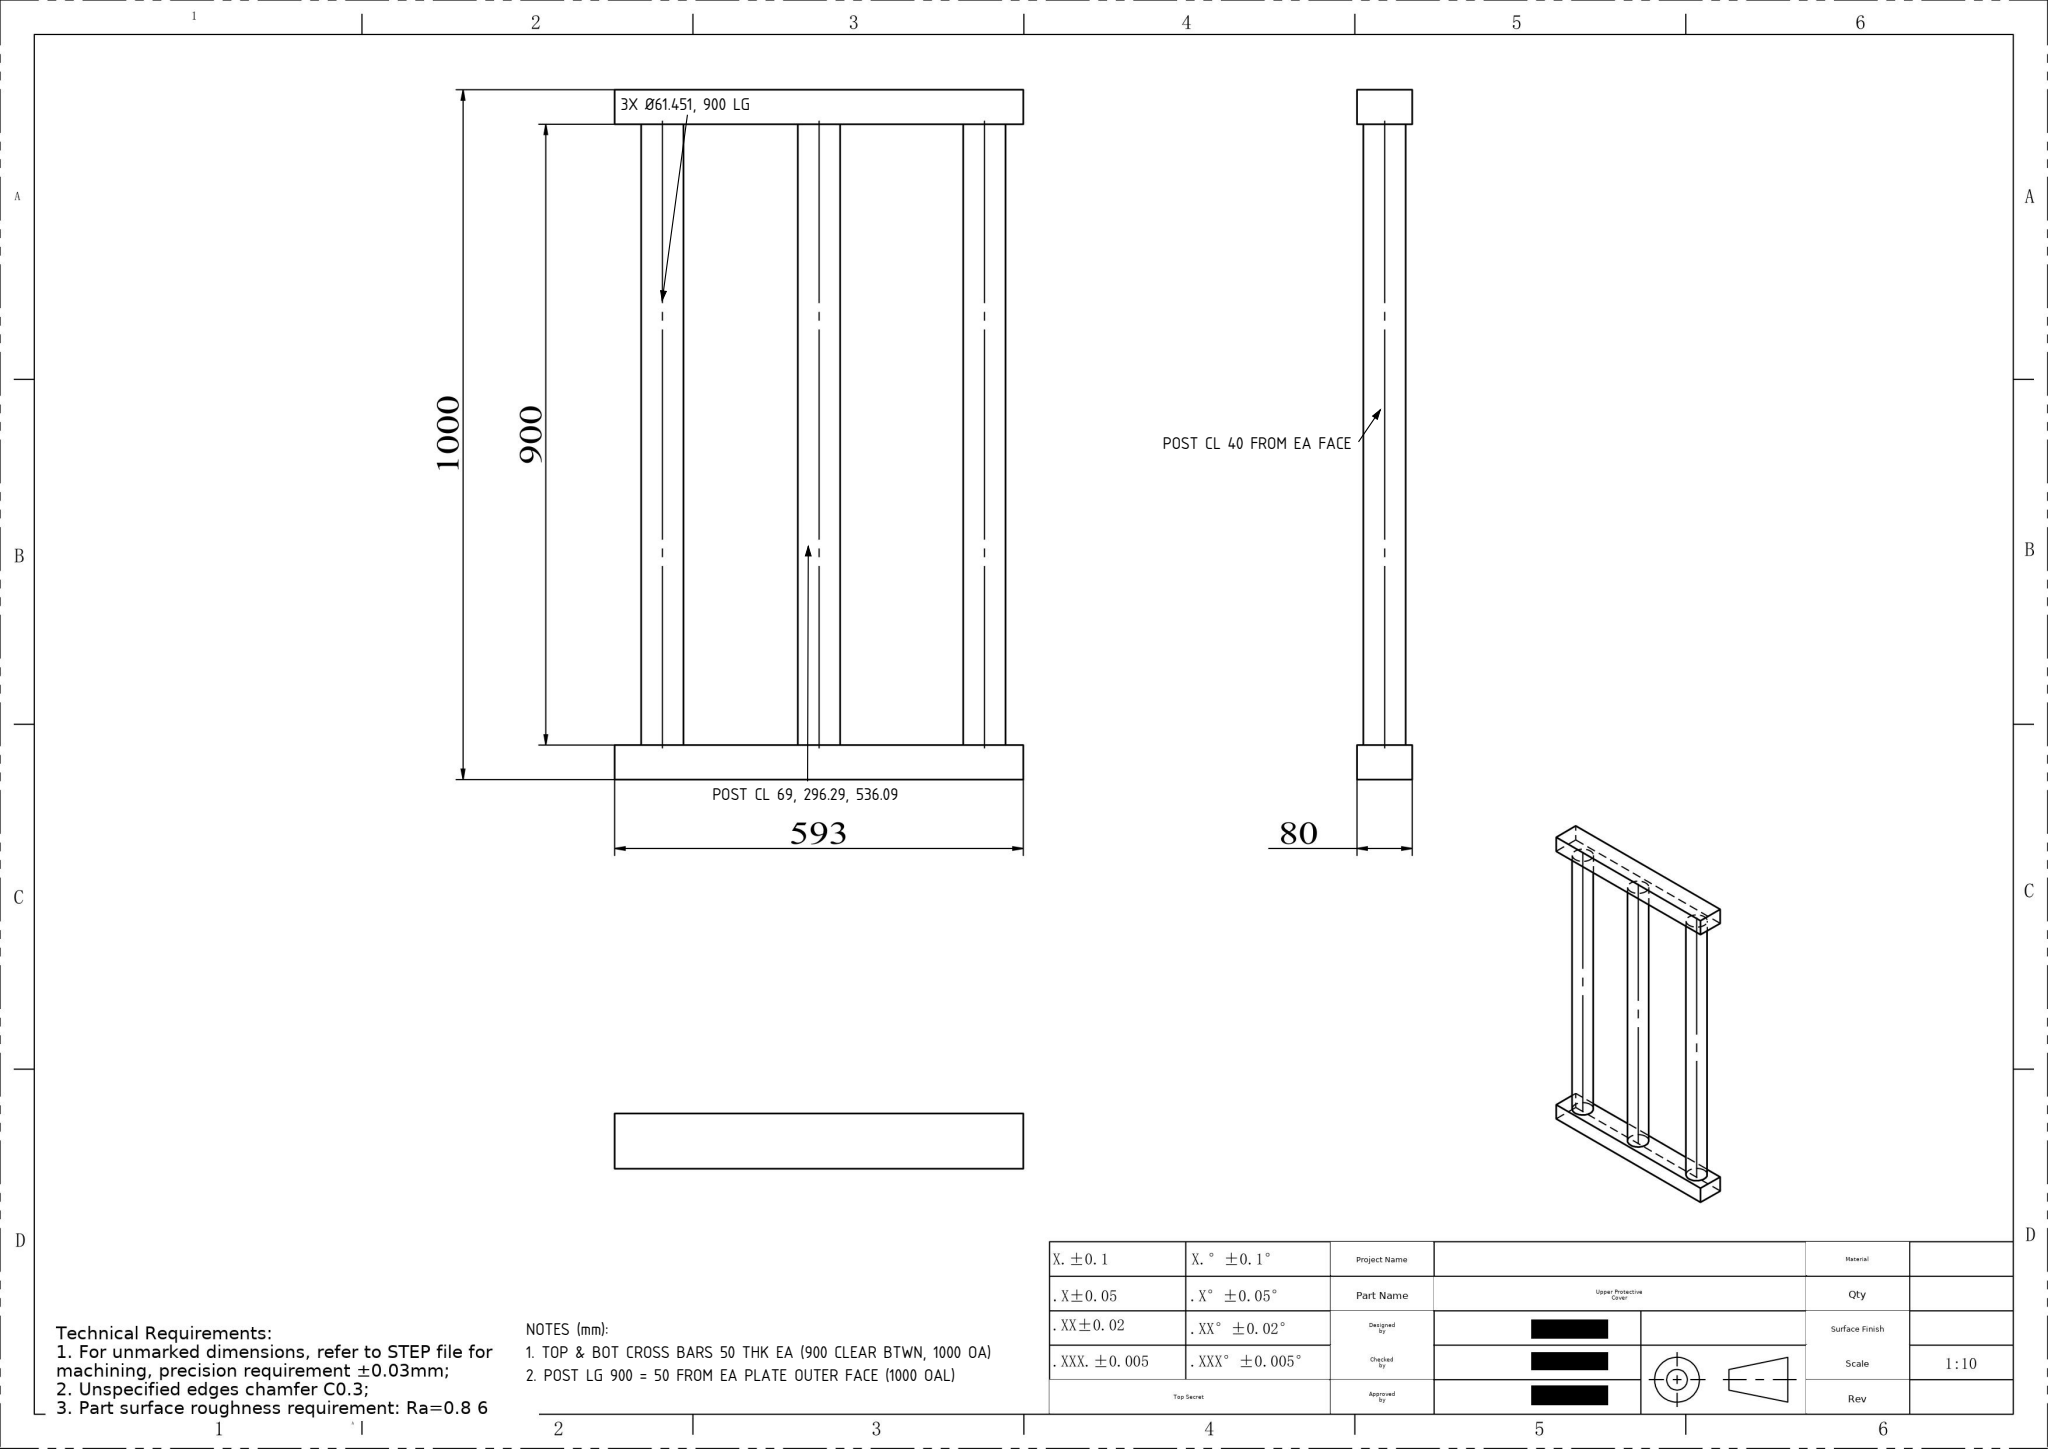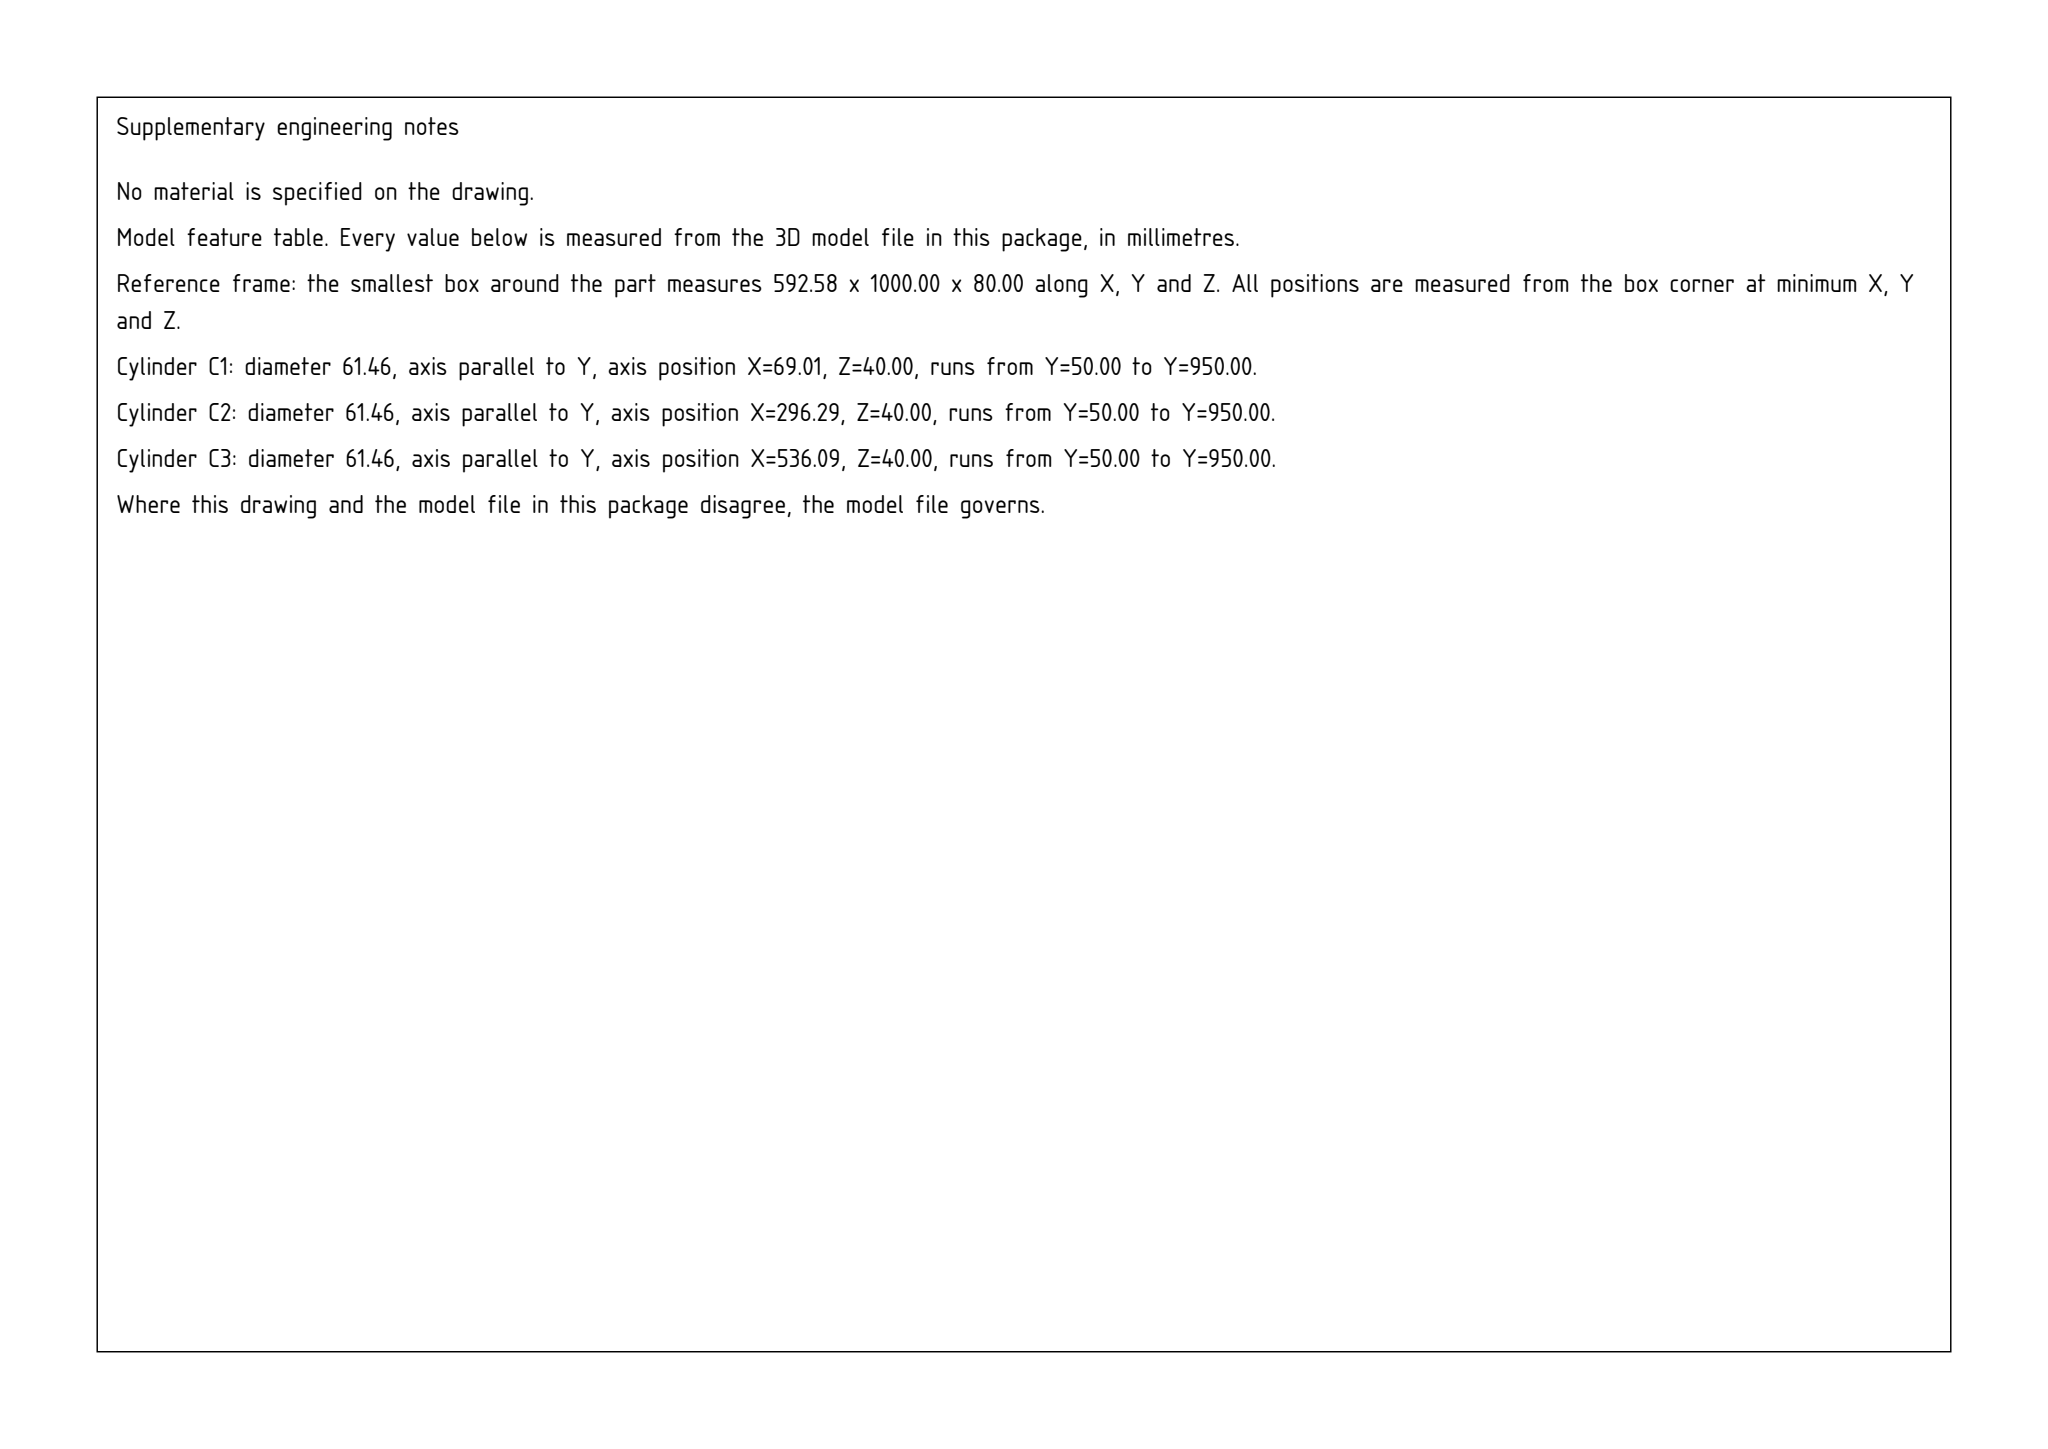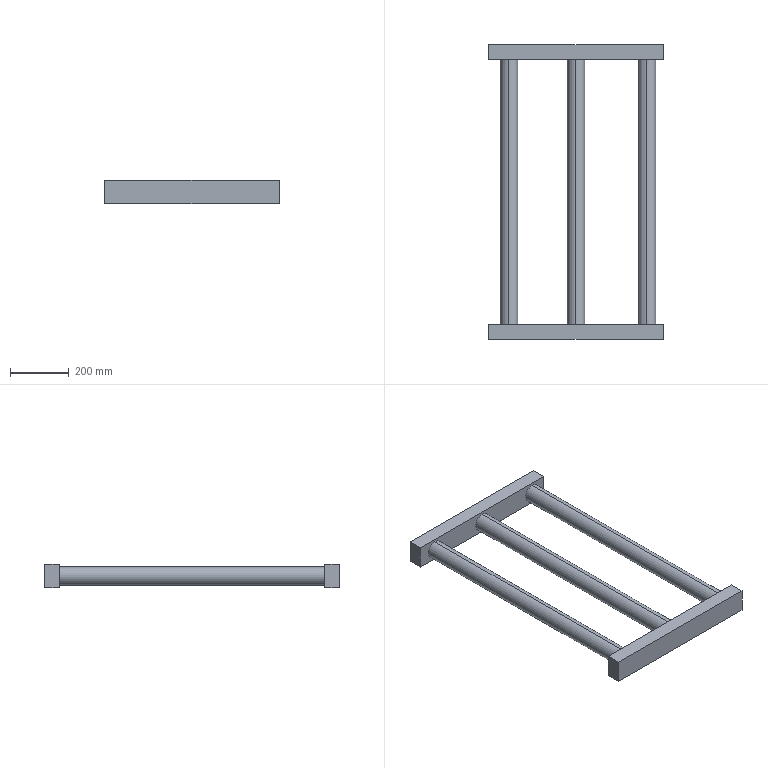Part | SolidWorks | mm | 1 solid | 18 faces | box 592.58 x 1000 x 80 mm | volume 12748485 mm3 | plane 12 | cylinder 6 | commonest cylinder face diameters 61.451 x6
Drawing notes:
TOP & BOT CROSS BARS 50 THK EA (900 CLEAR BTWN, 1000 OA) | from the solid: y-planes at 0/50 and 950/1000; rod length 900, bbox Y=1000
3X Ø61.451 VERT POSTS, 900 LG, FULL DEPTH BTWN END PLATES | from the solid: cylinders dia 61.451, axis y, length 900; plates y0-50 & y950-1000
POST CL FROM LH EDGE OF 593: 69, 296.29, 536.09 | from the solid: cylinder x positions 69.0, 296.29, 536.09 within bbox x=592.583
POST CL CENTERED IN 80 THK: 40 FROM EACH FACE | from the solid: cylinder z position 40.0; z planes at 0 and 80
POST LG 900 = 50 FROM EA PLATE OUTER FACE (1000 OAL) | from the solid: y planes 0, 50, 950, 1000; cylinder length 900
build123d program:
from build123d import *

# Parameters (mm, degrees)
SKETCH1_W             = 592.583
SKETCH1_H             = 50
BOSS_EXTRUDE1_DEPTH   = 80
BOSS_EXTRUDE1_2_DEPTH = 80
SKETCH2_R             = 30.726
BOSS_EXTRUDE2_DEPTH   = 950


with BuildPart() as part:
    # Sketch1 → Boss-Extrude1 (new body)
    with BuildSketch(Plane.XY):
        with Locations((-1944.166, 3836.21)):
            Rectangle(SKETCH1_W, SKETCH1_H)
    extrude(amount=BOSS_EXTRUDE1_DEPTH)



with BuildPart() as body_2:
    # Sketch1 → Boss-Extrude1 2 (new body)
    with BuildSketch(Plane.XY):
        with Locations((-1944.166, 2886.21)):
            Rectangle(SKETCH1_W, SKETCH1_H)
    extrude(amount=BOSS_EXTRUDE1_2_DEPTH)


with BuildPart() as part_1:
    add(part.part)

    add(body_2.part)  # Boss-Extrude2 merges body 2
    # Sketch2 → Boss-Extrude2 (add)
    with BuildSketch(Plane.XZ.offset(-3811.21)):
        with Locations(Location((-2171.453, 40, 0), (0, 0, 90))):
            Circle(SKETCH2_R)
        with Locations(Location((-1944.166, 40, 0), (0, 0, 90))):
            Circle(SKETCH2_R)
        with Locations(Location((-1704.372, 40, 0), (0, 0, 90))):
            Circle(SKETCH2_R)
    extrude(amount=BOSS_EXTRUDE2_DEPTH)


solid = part_1.part
STEP:
#1=CARTESIAN_POINT('',(-1704.372,2911.21,70.726));
#2=VERTEX_POINT('',#1);
#3=CARTESIAN_POINT('',(-1704.372,2911.21,9.274));
#4=VERTEX_POINT('',#3);
#5=CARTESIAN_POINT('',(-1704.372,2911.21,40.));
#6=DIRECTION('',(0.,1.,0.));
#7=DIRECTION('',(0.,0.,-1.));
#8=AXIS2_PLACEMENT_3D('',#5,#6,#7);
#9=CIRCLE('',#8,30.726);
#10=EDGE_CURVE('',#2,#4,#9,.T.);
#11=ORIENTED_EDGE('',*,*,#10,.T.);
#12=CARTESIAN_POINT('',(-1704.372,3811.21,9.274));
#13=VERTEX_POINT('',#12);
#14=CARTESIAN_POINT('',(-1704.372,2911.21,9.274));
#15=DIRECTION('',(0.,1.,0.));
#16=VECTOR('',#15,1000.);
#17=LINE('',#14,#16);
#18=EDGE_CURVE('',#4,#13,#17,.T.);
#19=ORIENTED_EDGE('',*,*,#18,.T.);
#20=CARTESIAN_POINT('',(-1704.372,3811.21,70.726));
#21=VERTEX_POINT('',#20);
#22=CARTESIAN_POINT('',(-1704.372,3811.21,40.));
#23=DIRECTION('',(0.,-1.,0.));
#24=DIRECTION('',(0.,0.,1.));
#25=AXIS2_PLACEMENT_3D('',#22,#23,#24);
#26=CIRCLE('',#25,30.726);
#27=EDGE_CURVE('',#13,#21,#26,.T.);
#28=ORIENTED_EDGE('',*,*,#27,.T.);
#29=CARTESIAN_POINT('',(-1704.372,2911.21,70.726));
#30=DIRECTION('',(0.,1.,0.));
#31=VECTOR('',#30,1000.);
#32=LINE('',#29,#31);
#33=EDGE_CURVE('',#2,#21,#32,.T.);
#34=ORIENTED_EDGE('',*,*,#33,.F.);
#35=EDGE_LOOP('',(#11,#19,#28,#34));
#36=FACE_OUTER_BOUND('',#35,.T.);
#37=CARTESIAN_POINT('',(-1704.372,2911.21,40.));
#38=DIRECTION('',(0.,1.,0.));
#39=DIRECTION('',(0.,0.,1.));
#40=AXIS2_PLACEMENT_3D('',#37,#38,#39);
#41=CYLINDRICAL_SURFACE('',#40,30.726);
#42=ADVANCED_FACE('',(#36),#41,.T.);
#43=CARTESIAN_POINT('',(-1944.166,2911.21,70.726));
#44=VERTEX_POINT('',#43);
#45=CARTESIAN_POINT('',(-1944.166,2911.21,9.274));
#46=VERTEX_POINT('',#45);
#47=CARTESIAN_POINT('',(-1944.166,2911.21,40.));
#48=DIRECTION('',(0.,1.,0.));
#49=DIRECTION('',(0.,0.,-1.));
#50=AXIS2_PLACEMENT_3D('',#47,#48,#49);
#51=CIRCLE('',#50,30.726);
#52=EDGE_CURVE('',#44,#46,#51,.T.);
#53=ORIENTED_EDGE('',*,*,#52,.T.);
#54=CARTESIAN_POINT('',(-1944.166,3811.21,9.274));
#55=VERTEX_POINT('',#54);
#56=CARTESIAN_POINT('',(-1944.166,2911.21,9.274));
#57=DIRECTION('',(0.,1.,0.));
#58=VECTOR('',#57,1000.);
#59=LINE('',#56,#58);
#60=EDGE_CURVE('',#46,#55,#59,.T.);
#61=ORIENTED_EDGE('',*,*,#60,.T.);
#62=CARTESIAN_POINT('',(-1944.166,3811.21,70.726));
#63=VERTEX_POINT('',#62);
#64=CARTESIAN_POINT('',(-1944.166,3811.21,40.));
#65=DIRECTION('',(0.,-1.,0.));
#66=DIRECTION('',(0.,0.,1.));
#67=AXIS2_PLACEMENT_3D('',#64,#65,#66);
#68=CIRCLE('',#67,30.726);
#69=EDGE_CURVE('',#55,#63,#68,.T.);
#70=ORIENTED_EDGE('',*,*,#69,.T.);
#71=CARTESIAN_POINT('',(-1944.166,2911.21,70.726));
#72=DIRECTION('',(0.,1.,0.));
#73=VECTOR('',#72,1000.);
#74=LINE('',#71,#73);
#75=EDGE_CURVE('',#44,#63,#74,.T.);
#76=ORIENTED_EDGE('',*,*,#75,.F.);
#77=EDGE_LOOP('',(#53,#61,#70,#76));
#78=FACE_OUTER_BOUND('',#77,.T.);
#79=CARTESIAN_POINT('',(-1944.166,2911.21,40.));
#80=DIRECTION('',(0.,1.,0.));
#81=DIRECTION('',(0.,0.,1.));
#82=AXIS2_PLACEMENT_3D('',#79,#80,#81);
#83=CYLINDRICAL_SURFACE('',#82,30.726);
#84=ADVANCED_FACE('',(#78),#83,.T.);
#85=CARTESIAN_POINT('',(-2171.453,2911.21,9.274));
#86=VERTEX_POINT('',#85);
#87=CARTESIAN_POINT('',(-2171.453,2911.21,70.726));
#88=VERTEX_POINT('',#87);
#89=CARTESIAN_POINT('',(-2171.453,2911.21,40.));
#90=DIRECTION('',(0.,-1.,0.));
#91=DIRECTION('',(0.,0.,-1.));
#92=AXIS2_PLACEMENT_3D('',#89,#90,#91);
#93=CIRCLE('',#92,30.726);
#94=EDGE_CURVE('',#86,#88,#93,.T.);
#95=ORIENTED_EDGE('',*,*,#94,.F.);
#96=CARTESIAN_POINT('',(-2171.453,3811.21,9.274));
#97=VERTEX_POINT('',#96);
#98=CARTESIAN_POINT('',(-2171.453,2911.21,9.274));
#99=DIRECTION('',(0.,1.,0.));
#100=VECTOR('',#99,1000.);
#101=LINE('',#98,#100);
#102=EDGE_CURVE('',#86,#97,#101,.T.);
#103=ORIENTED_EDGE('',*,*,#102,.T.);
#104=CARTESIAN_POINT('',(-2171.453,3811.21,70.726));
#105=VERTEX_POINT('',#104);
#106=CARTESIAN_POINT('',(-2171.453,3811.21,40.));
#107=DIRECTION('',(0.,-1.,0.));
#108=DIRECTION('',(0.,0.,1.));
#109=AXIS2_PLACEMENT_3D('',#106,#107,#108);
#110=CIRCLE('',#109,30.726);
#111=EDGE_CURVE('',#97,#105,#110,.T.);
#112=ORIENTED_EDGE('',*,*,#111,.T.);
#113=CARTESIAN_POINT('',(-2171.453,2911.21,70.726));
#114=DIRECTION('',(0.,1.,0.));
#115=VECTOR('',#114,1000.);
#116=LINE('',#113,#115);
#117=EDGE_CURVE('',#88,#105,#116,.T.);
#118=ORIENTED_EDGE('',*,*,#117,.F.);
#119=EDGE_LOOP('',(#95,#103,#112,#118));
#120=FACE_OUTER_BOUND('',#119,.T.);
#121=CARTESIAN_POINT('',(-2171.453,2911.21,40.));
#122=DIRECTION('',(0.,1.,0.));
#123=DIRECTION('',(0.,0.,1.));
#124=AXIS2_PLACEMENT_3D('',#121,#122,#123);
#125=CYLINDRICAL_SURFACE('',#124,30.726);
#126=ADVANCED_FACE('',(#120),#125,.T.);
#127=CARTESIAN_POINT('',(-2240.457,3861.21,0.));
#128=VERTEX_POINT('',#127);
#129=CARTESIAN_POINT('',(-2240.457,3811.21,0.));
#130=VERTEX_POINT('',#129);
#131=CARTESIAN_POINT('',(-2240.457,3861.21,0.));
#132=DIRECTION('',(0.,-1.,0.));
#133=VECTOR('',#132,1000.);
#134=LINE('',#131,#133);
#135=EDGE_CURVE('',#128,#130,#134,.T.);
#136=ORIENTED_EDGE('',*,*,#135,.T.);
#137=CARTESIAN_POINT('',(-2240.457,3811.21,80.));
#138=VERTEX_POINT('',#137);
#139=CARTESIAN_POINT('',(-2240.457,3811.21,80.));
#140=DIRECTION('',(0.,0.,-1.));
#141=VECTOR('',#140,1000.);
#142=LINE('',#139,#141);
#143=EDGE_CURVE('',#138,#130,#142,.T.);
#144=ORIENTED_EDGE('',*,*,#143,.F.);
#145=CARTESIAN_POINT('',(-2240.457,3861.21,80.));
#146=VERTEX_POINT('',#145);
#147=CARTESIAN_POINT('',(-2240.457,3861.21,80.));
#148=DIRECTION('',(0.,-1.,0.));
#149=VECTOR('',#148,1000.);
#150=LINE('',#147,#149);
#151=EDGE_CURVE('',#146,#138,#150,.T.);
#152=ORIENTED_EDGE('',*,*,#151,.F.);
#153=CARTESIAN_POINT('',(-2240.457,3861.21,80.));
#154=DIRECTION('',(0.,0.,-1.));
#155=VECTOR('',#154,1000.);
#156=LINE('',#153,#155);
#157=EDGE_CURVE('',#146,#128,#156,.T.);
#158=ORIENTED_EDGE('',*,*,#157,.T.);
#159=EDGE_LOOP('',(#136,#144,#152,#158));
#160=FACE_OUTER_BOUND('',#159,.T.);
#161=CARTESIAN_POINT('',(-2240.457,3861.21,80.));
#162=DIRECTION('',(1.,0.,0.));
#163=DIRECTION('',(0.,0.,-1.));
#164=AXIS2_PLACEMENT_3D('',#161,#162,#163);
#165=PLANE('',#164);
#166=ADVANCED_FACE('',(#160),#165,.F.);
#167=CARTESIAN_POINT('',(-1704.372,3811.21,40.));
#168=DIRECTION('',(0.,-1.,0.));
#169=DIRECTION('',(0.,0.,1.));
#170=AXIS2_PLACEMENT_3D('',#167,#168,#169);
#171=CIRCLE('',#170,30.726);
#172=EDGE_CURVE('',#21,#13,#171,.T.);
#173=ORIENTED_EDGE('',*,*,#172,.F.);
#174=ORIENTED_EDGE('',*,*,#27,.F.);
#175=EDGE_LOOP('',(#173,#174));
#176=FACE_BOUND('',#175,.T.);
#177=CARTESIAN_POINT('',(-1944.166,3811.21,40.));
#178=DIRECTION('',(0.,-1.,0.));
#179=DIRECTION('',(0.,0.,1.));
#180=AXIS2_PLACEMENT_3D('',#177,#178,#179);
#181=CIRCLE('',#180,30.726);
#182=EDGE_CURVE('',#63,#55,#181,.T.);
#183=ORIENTED_EDGE('',*,*,#182,.F.);
#184=ORIENTED_EDGE('',*,*,#69,.F.);
#185=EDGE_LOOP('',(#183,#184));
#186=FACE_BOUND('',#185,.T.);
#187=CARTESIAN_POINT('',(-2171.453,3811.21,40.));
#188=DIRECTION('',(0.,-1.,0.));
#189=DIRECTION('',(0.,0.,1.));
#190=AXIS2_PLACEMENT_3D('',#187,#188,#189);
#191=CIRCLE('',#190,30.726);
#192=EDGE_CURVE('',#105,#97,#191,.T.);
#193=ORIENTED_EDGE('',*,*,#192,.F.);
#194=ORIENTED_EDGE('',*,*,#111,.F.);
#195=EDGE_LOOP('',(#193,#194));
#196=FACE_BOUND('',#195,.T.);
#197=CARTESIAN_POINT('',(-1647.875,3811.21,0.));
#198=VERTEX_POINT('',#197);
#199=CARTESIAN_POINT('',(-2240.457,3811.21,0.));
#200=DIRECTION('',(1.,0.,0.));
#201=VECTOR('',#200,1000.);
#202=LINE('',#199,#201);
#203=EDGE_CURVE('',#130,#198,#202,.T.);
#204=ORIENTED_EDGE('',*,*,#203,.T.);
#205=CARTESIAN_POINT('',(-1647.875,3811.21,80.));
#206=VERTEX_POINT('',#205);
#207=CARTESIAN_POINT('',(-1647.875,3811.21,80.));
#208=DIRECTION('',(0.,0.,-1.));
#209=VECTOR('',#208,1000.);
#210=LINE('',#207,#209);
#211=EDGE_CURVE('',#206,#198,#210,.T.);
#212=ORIENTED_EDGE('',*,*,#211,.F.);
#213=CARTESIAN_POINT('',(-2240.457,3811.21,80.));
#214=DIRECTION('',(1.,0.,0.));
#215=VECTOR('',#214,1000.);
#216=LINE('',#213,#215);
#217=EDGE_CURVE('',#138,#206,#216,.T.);
#218=ORIENTED_EDGE('',*,*,#217,.F.);
#219=ORIENTED_EDGE('',*,*,#143,.T.);
#220=EDGE_LOOP('',(#204,#212,#218,#219));
#221=FACE_OUTER_BOUND('',#220,.T.);
#222=CARTESIAN_POINT('',(-2240.457,3811.21,80.));
#223=DIRECTION('',(0.,1.,0.));
#224=DIRECTION('',(0.,0.,1.));
#225=AXIS2_PLACEMENT_3D('',#222,#223,#224);
#226=PLANE('',#225);
#227=ADVANCED_FACE('',(#176,#186,#196,#221),#226,.F.);
#228=CARTESIAN_POINT('',(-1647.875,3861.21,0.));
#229=VERTEX_POINT('',#228);
#230=CARTESIAN_POINT('',(-1647.875,3861.21,0.));
#231=DIRECTION('',(0.,1.,0.));
#232=VECTOR('',#231,1000.);
#233=LINE('',#230,#232);
#234=EDGE_CURVE('',#198,#229,#233,.T.);
#235=ORIENTED_EDGE('',*,*,#234,.T.);
#236=CARTESIAN_POINT('',(-1647.875,3861.21,80.));
#237=VERTEX_POINT('',#236);
#238=CARTESIAN_POINT('',(-1647.875,3861.21,80.));
#239=DIRECTION('',(0.,0.,-1.));
#240=VECTOR('',#239,1000.);
#241=LINE('',#238,#240);
#242=EDGE_CURVE('',#237,#229,#241,.T.);
#243=ORIENTED_EDGE('',*,*,#242,.F.);
#244=CARTESIAN_POINT('',(-1647.875,3861.21,80.));
#245=DIRECTION('',(0.,1.,0.));
#246=VECTOR('',#245,1000.);
#247=LINE('',#244,#246);
#248=EDGE_CURVE('',#206,#237,#247,.T.);
#249=ORIENTED_EDGE('',*,*,#248,.F.);
#250=ORIENTED_EDGE('',*,*,#211,.T.);
#251=EDGE_LOOP('',(#235,#243,#249,#250));
#252=FACE_OUTER_BOUND('',#251,.T.);
#253=CARTESIAN_POINT('',(-1647.875,3861.21,80.));
#254=DIRECTION('',(-1.,0.,0.));
#255=DIRECTION('',(0.,0.,1.));
#256=AXIS2_PLACEMENT_3D('',#253,#254,#255);
#257=PLANE('',#256);
#258=ADVANCED_FACE('',(#252),#257,.F.);
#259=CARTESIAN_POINT('',(-2240.457,3861.21,0.));
#260=DIRECTION('',(-1.,0.,0.));
#261=VECTOR('',#260,1000.);
#262=LINE('',#259,#261);
#263=EDGE_CURVE('',#229,#128,#262,.T.);
#264=ORIENTED_EDGE('',*,*,#263,.T.);
#265=ORIENTED_EDGE('',*,*,#157,.F.);
#266=CARTESIAN_POINT('',(-2240.457,3861.21,80.));
#267=DIRECTION('',(-1.,0.,0.));
#268=VECTOR('',#267,1000.);
#269=LINE('',#266,#268);
#270=EDGE_CURVE('',#237,#146,#269,.T.);
#271=ORIENTED_EDGE('',*,*,#270,.F.);
#272=ORIENTED_EDGE('',*,*,#242,.T.);
#273=EDGE_LOOP('',(#264,#265,#271,#272));
#274=FACE_OUTER_BOUND('',#273,.T.);
#275=CARTESIAN_POINT('',(-2240.457,3861.21,80.));
#276=DIRECTION('',(0.,-1.,0.));
#277=DIRECTION('',(0.,0.,-1.));
#278=AXIS2_PLACEMENT_3D('',#275,#276,#277);
#279=PLANE('',#278);
#280=ADVANCED_FACE('',(#274),#279,.F.);
#281=ORIENTED_EDGE('',*,*,#151,.T.);
#282=ORIENTED_EDGE('',*,*,#217,.T.);
#283=ORIENTED_EDGE('',*,*,#248,.T.);
#284=ORIENTED_EDGE('',*,*,#270,.T.);
#285=EDGE_LOOP('',(#281,#282,#283,#284));
#286=FACE_OUTER_BOUND('',#285,.T.);
#287=CARTESIAN_POINT('',(0.,0.,80.));
#288=DIRECTION('',(0.,0.,1.));
#289=DIRECTION('',(1.,0.,0.));
#290=AXIS2_PLACEMENT_3D('',#287,#288,#289);
#291=PLANE('',#290);
#292=ADVANCED_FACE('',(#286),#291,.T.);
#293=ORIENTED_EDGE('',*,*,#135,.F.);
#294=ORIENTED_EDGE('',*,*,#263,.F.);
#295=ORIENTED_EDGE('',*,*,#234,.F.);
#296=ORIENTED_EDGE('',*,*,#203,.F.);
#297=EDGE_LOOP('',(#293,#294,#295,#296));
#298=FACE_OUTER_BOUND('',#297,.T.);
#299=CARTESIAN_POINT('',(0.,0.,0.));
#300=DIRECTION('',(0.,0.,1.));
#301=DIRECTION('',(1.,0.,0.));
#302=AXIS2_PLACEMENT_3D('',#299,#300,#301);
#303=PLANE('',#302);
#304=ADVANCED_FACE('',(#298),#303,.F.);
#305=ORIENTED_EDGE('',*,*,#102,.F.);
#306=CARTESIAN_POINT('',(-2171.453,2911.21,40.));
#307=DIRECTION('',(0.,-1.,0.));
#308=DIRECTION('',(0.,0.,-1.));
#309=AXIS2_PLACEMENT_3D('',#306,#307,#308);
#310=CIRCLE('',#309,30.726);
#311=EDGE_CURVE('',#88,#86,#310,.T.);
#312=ORIENTED_EDGE('',*,*,#311,.F.);
#313=ORIENTED_EDGE('',*,*,#117,.T.);
#314=ORIENTED_EDGE('',*,*,#192,.T.);
#315=EDGE_LOOP('',(#305,#312,#313,#314));
#316=FACE_OUTER_BOUND('',#315,.T.);
#317=CARTESIAN_POINT('',(-2171.453,2911.21,40.));
#318=DIRECTION('',(0.,1.,0.));
#319=DIRECTION('',(0.,0.,1.));
#320=AXIS2_PLACEMENT_3D('',#317,#318,#319);
#321=CYLINDRICAL_SURFACE('',#320,30.726);
#322=ADVANCED_FACE('',(#316),#321,.T.);
#323=CARTESIAN_POINT('',(-2240.457,2911.21,0.));
#324=VERTEX_POINT('',#323);
#325=CARTESIAN_POINT('',(-2240.457,2861.21,0.));
#326=VERTEX_POINT('',#325);
#327=CARTESIAN_POINT('',(-2240.457,2861.21,0.));
#328=DIRECTION('',(0.,-1.,0.));
#329=VECTOR('',#328,1000.);
#330=LINE('',#327,#329);
#331=EDGE_CURVE('',#324,#326,#330,.T.);
#332=ORIENTED_EDGE('',*,*,#331,.T.);
#333=CARTESIAN_POINT('',(-2240.457,2861.21,80.));
#334=VERTEX_POINT('',#333);
#335=CARTESIAN_POINT('',(-2240.457,2861.21,80.));
#336=DIRECTION('',(0.,0.,-1.));
#337=VECTOR('',#336,1000.);
#338=LINE('',#335,#337);
#339=EDGE_CURVE('',#334,#326,#338,.T.);
#340=ORIENTED_EDGE('',*,*,#339,.F.);
#341=CARTESIAN_POINT('',(-2240.457,2911.21,80.));
#342=VERTEX_POINT('',#341);
#343=CARTESIAN_POINT('',(-2240.457,2861.21,80.));
#344=DIRECTION('',(0.,-1.,0.));
#345=VECTOR('',#344,1000.);
#346=LINE('',#343,#345);
#347=EDGE_CURVE('',#342,#334,#346,.T.);
#348=ORIENTED_EDGE('',*,*,#347,.F.);
#349=CARTESIAN_POINT('',(-2240.457,2911.21,80.));
#350=DIRECTION('',(0.,0.,-1.));
#351=VECTOR('',#350,1000.);
#352=LINE('',#349,#351);
#353=EDGE_CURVE('',#342,#324,#352,.T.);
#354=ORIENTED_EDGE('',*,*,#353,.T.);
#355=EDGE_LOOP('',(#332,#340,#348,#354));
#356=FACE_OUTER_BOUND('',#355,.T.);
#357=CARTESIAN_POINT('',(-2240.457,2861.21,80.));
#358=DIRECTION('',(1.,0.,0.));
#359=DIRECTION('',(0.,0.,-1.));
#360=AXIS2_PLACEMENT_3D('',#357,#358,#359);
#361=PLANE('',#360);
#362=ADVANCED_FACE('',(#356),#361,.F.);
#363=CARTESIAN_POINT('',(-1647.875,2861.21,0.));
#364=VERTEX_POINT('',#363);
#365=CARTESIAN_POINT('',(-2240.457,2861.21,0.));
#366=DIRECTION('',(1.,0.,0.));
#367=VECTOR('',#366,1000.);
#368=LINE('',#365,#367);
#369=EDGE_CURVE('',#326,#364,#368,.T.);
#370=ORIENTED_EDGE('',*,*,#369,.T.);
#371=CARTESIAN_POINT('',(-1647.875,2861.21,80.));
#372=VERTEX_POINT('',#371);
#373=CARTESIAN_POINT('',(-1647.875,2861.21,80.));
#374=DIRECTION('',(0.,0.,-1.));
#375=VECTOR('',#374,1000.);
#376=LINE('',#373,#375);
#377=EDGE_CURVE('',#372,#364,#376,.T.);
#378=ORIENTED_EDGE('',*,*,#377,.F.);
#379=CARTESIAN_POINT('',(-2240.457,2861.21,80.));
#380=DIRECTION('',(1.,0.,0.));
#381=VECTOR('',#380,1000.);
#382=LINE('',#379,#381);
#383=EDGE_CURVE('',#334,#372,#382,.T.);
#384=ORIENTED_EDGE('',*,*,#383,.F.);
#385=ORIENTED_EDGE('',*,*,#339,.T.);
#386=EDGE_LOOP('',(#370,#378,#384,#385));
#387=FACE_OUTER_BOUND('',#386,.T.);
#388=CARTESIAN_POINT('',(-2240.457,2861.21,80.));
#389=DIRECTION('',(0.,1.,0.));
#390=DIRECTION('',(0.,0.,1.));
#391=AXIS2_PLACEMENT_3D('',#388,#389,#390);
#392=PLANE('',#391);
#393=ADVANCED_FACE('',(#387),#392,.F.);
#394=CARTESIAN_POINT('',(-1647.875,2911.21,0.));
#395=VERTEX_POINT('',#394);
#396=CARTESIAN_POINT('',(-1647.875,2861.21,0.));
#397=DIRECTION('',(0.,1.,0.));
#398=VECTOR('',#397,1000.);
#399=LINE('',#396,#398);
#400=EDGE_CURVE('',#364,#395,#399,.T.);
#401=ORIENTED_EDGE('',*,*,#400,.T.);
#402=CARTESIAN_POINT('',(-1647.875,2911.21,80.));
#403=VERTEX_POINT('',#402);
#404=CARTESIAN_POINT('',(-1647.875,2911.21,80.));
#405=DIRECTION('',(0.,0.,-1.));
#406=VECTOR('',#405,1000.);
#407=LINE('',#404,#406);
#408=EDGE_CURVE('',#403,#395,#407,.T.);
#409=ORIENTED_EDGE('',*,*,#408,.F.);
#410=CARTESIAN_POINT('',(-1647.875,2861.21,80.));
#411=DIRECTION('',(0.,1.,0.));
#412=VECTOR('',#411,1000.);
#413=LINE('',#410,#412);
#414=EDGE_CURVE('',#372,#403,#413,.T.);
#415=ORIENTED_EDGE('',*,*,#414,.F.);
#416=ORIENTED_EDGE('',*,*,#377,.T.);
#417=EDGE_LOOP('',(#401,#409,#415,#416));
#418=FACE_OUTER_BOUND('',#417,.T.);
#419=CARTESIAN_POINT('',(-1647.875,2861.21,80.));
#420=DIRECTION('',(-1.,0.,0.));
#421=DIRECTION('',(0.,0.,1.));
#422=AXIS2_PLACEMENT_3D('',#419,#420,#421);
#423=PLANE('',#422);
#424=ADVANCED_FACE('',(#418),#423,.F.);
#425=ORIENTED_EDGE('',*,*,#10,.F.);
#426=CARTESIAN_POINT('',(-1704.372,2911.21,40.));
#427=DIRECTION('',(0.,1.,0.));
#428=DIRECTION('',(0.,0.,-1.));
#429=AXIS2_PLACEMENT_3D('',#426,#427,#428);
#430=CIRCLE('',#429,30.726);
#431=EDGE_CURVE('',#4,#2,#430,.T.);
#432=ORIENTED_EDGE('',*,*,#431,.F.);
#433=EDGE_LOOP('',(#425,#432));
#434=FACE_BOUND('',#433,.T.);
#435=ORIENTED_EDGE('',*,*,#52,.F.);
#436=CARTESIAN_POINT('',(-1944.166,2911.21,40.));
#437=DIRECTION('',(0.,1.,0.));
#438=DIRECTION('',(0.,0.,-1.));
#439=AXIS2_PLACEMENT_3D('',#436,#437,#438);
#440=CIRCLE('',#439,30.726);
#441=EDGE_CURVE('',#46,#44,#440,.T.);
#442=ORIENTED_EDGE('',*,*,#441,.F.);
#443=EDGE_LOOP('',(#435,#442));
#444=FACE_BOUND('',#443,.T.);
#445=ORIENTED_EDGE('',*,*,#311,.T.);
#446=ORIENTED_EDGE('',*,*,#94,.T.);
#447=EDGE_LOOP('',(#445,#446));
#448=FACE_BOUND('',#447,.T.);
#449=CARTESIAN_POINT('',(-2240.457,2911.21,0.));
#450=DIRECTION('',(-1.,0.,0.));
#451=VECTOR('',#450,1000.);
#452=LINE('',#449,#451);
#453=EDGE_CURVE('',#395,#324,#452,.T.);
#454=ORIENTED_EDGE('',*,*,#453,.T.);
#455=ORIENTED_EDGE('',*,*,#353,.F.);
#456=CARTESIAN_POINT('',(-2240.457,2911.21,80.));
#457=DIRECTION('',(-1.,0.,0.));
#458=VECTOR('',#457,1000.);
#459=LINE('',#456,#458);
#460=EDGE_CURVE('',#403,#342,#459,.T.);
#461=ORIENTED_EDGE('',*,*,#460,.F.);
#462=ORIENTED_EDGE('',*,*,#408,.T.);
#463=EDGE_LOOP('',(#454,#455,#461,#462));
#464=FACE_OUTER_BOUND('',#463,.T.);
#465=CARTESIAN_POINT('',(-2240.457,2911.21,80.));
#466=DIRECTION('',(0.,-1.,0.));
#467=DIRECTION('',(0.,0.,-1.));
#468=AXIS2_PLACEMENT_3D('',#465,#466,#467);
#469=PLANE('',#468);
#470=ADVANCED_FACE('',(#434,#444,#448,#464),#469,.F.);
#471=ORIENTED_EDGE('',*,*,#347,.T.);
#472=ORIENTED_EDGE('',*,*,#383,.T.);
#473=ORIENTED_EDGE('',*,*,#414,.T.);
#474=ORIENTED_EDGE('',*,*,#460,.T.);
#475=EDGE_LOOP('',(#471,#472,#473,#474));
#476=FACE_OUTER_BOUND('',#475,.T.);
#477=CARTESIAN_POINT('',(0.,0.,80.));
#478=DIRECTION('',(0.,0.,-1.));
#479=DIRECTION('',(-1.,0.,0.));
#480=AXIS2_PLACEMENT_3D('',#477,#478,#479);
#481=PLANE('',#480);
#482=ADVANCED_FACE('',(#476),#481,.F.);
#483=ORIENTED_EDGE('',*,*,#331,.F.);
#484=ORIENTED_EDGE('',*,*,#453,.F.);
#485=ORIENTED_EDGE('',*,*,#400,.F.);
#486=ORIENTED_EDGE('',*,*,#369,.F.);
#487=EDGE_LOOP('',(#483,#484,#485,#486));
#488=FACE_OUTER_BOUND('',#487,.T.);
#489=CARTESIAN_POINT('',(0.,0.,0.));
#490=DIRECTION('',(0.,0.,-1.));
#491=DIRECTION('',(-1.,0.,0.));
#492=AXIS2_PLACEMENT_3D('',#489,#490,#491);
#493=PLANE('',#492);
#494=ADVANCED_FACE('',(#488),#493,.T.);
#495=ORIENTED_EDGE('',*,*,#60,.F.);
#496=ORIENTED_EDGE('',*,*,#441,.T.);
#497=ORIENTED_EDGE('',*,*,#75,.T.);
#498=ORIENTED_EDGE('',*,*,#182,.T.);
#499=EDGE_LOOP('',(#495,#496,#497,#498));
#500=FACE_OUTER_BOUND('',#499,.T.);
#501=CARTESIAN_POINT('',(-1944.166,2911.21,40.));
#502=DIRECTION('',(0.,1.,0.));
#503=DIRECTION('',(0.,0.,1.));
#504=AXIS2_PLACEMENT_3D('',#501,#502,#503);
#505=CYLINDRICAL_SURFACE('',#504,30.726);
#506=ADVANCED_FACE('',(#500),#505,.T.);
#507=ORIENTED_EDGE('',*,*,#18,.F.);
#508=ORIENTED_EDGE('',*,*,#431,.T.);
#509=ORIENTED_EDGE('',*,*,#33,.T.);
#510=ORIENTED_EDGE('',*,*,#172,.T.);
#511=EDGE_LOOP('',(#507,#508,#509,#510));
#512=FACE_OUTER_BOUND('',#511,.T.);
#513=CARTESIAN_POINT('',(-1704.372,2911.21,40.));
#514=DIRECTION('',(0.,1.,0.));
#515=DIRECTION('',(0.,0.,1.));
#516=AXIS2_PLACEMENT_3D('',#513,#514,#515);
#517=CYLINDRICAL_SURFACE('',#516,30.726);
#518=ADVANCED_FACE('',(#512),#517,.T.);
#519=CLOSED_SHELL('',(#42,#84,#126,#166,#227,#258,#280,#292,#304,#322,#362,#393,#424,#470,#482,#494,#506,#518));
#520=MANIFOLD_SOLID_BREP('',#519);
#521=CARTESIAN_POINT('',(0.,0.,0.));
#522=DIRECTION('',(0.,0.,1.));
#523=DIRECTION('',(1.,0.,0.));
#524=AXIS2_PLACEMENT_3D('',#521,#522,#523);
#525=(LENGTH_UNIT()NAMED_UNIT(*)SI_UNIT(.MILLI.,.METRE.));
#526=UNCERTAINTY_MEASURE_WITH_UNIT(LENGTH_MEASURE(0.00001),#525,'','');
#527=(NAMED_UNIT(*)PLANE_ANGLE_UNIT()SI_UNIT($,.RADIAN.));
#528=(NAMED_UNIT(*)SI_UNIT($,.STERADIAN.)SOLID_ANGLE_UNIT());
#529=(GEOMETRIC_REPRESENTATION_CONTEXT(3)GLOBAL_UNCERTAINTY_ASSIGNED_CONTEXT((#526))GLOBAL_UNIT_ASSIGNED_CONTEXT((#525,#527,#528))REPRESENTATION_CONTEXT('',''));
#530=ADVANCED_BREP_SHAPE_REPRESENTATION('',(#520,#524),#529);